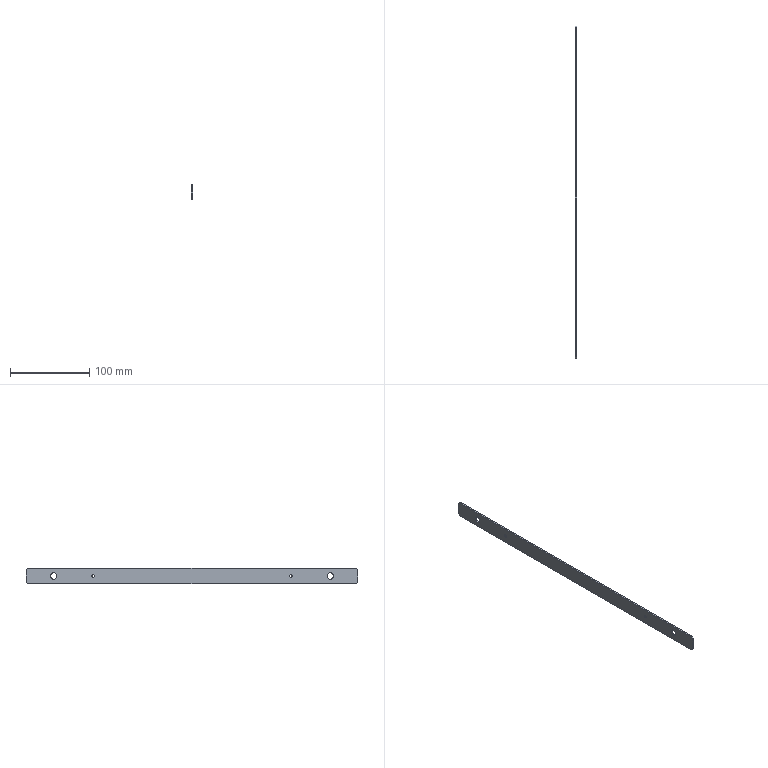Component | SolidWorks | 10-15A-1 | 1 solid | 18 faces | box 2 x 420 x 20 mm | volume 16549 mm3 | plane 10 | cylinder 8 | commonest cylinder face diameters 3.3 x4 8 x4
STEP:
#1=COLOUR_RGB('',0.7922,0.8196,0.9333);
#2=FILL_AREA_STYLE_COLOUR('',#1);
#3=FILL_AREA_STYLE('',(#2));
#4=SURFACE_STYLE_FILL_AREA(#3);
#5=SURFACE_SIDE_STYLE('',(#4));
#6=SURFACE_STYLE_USAGE(.BOTH.,#5);
#7=PRESENTATION_STYLE_ASSIGNMENT((#6));
#8=CARTESIAN_POINT('',(-17.615,14.849,0.8524));
#9=VERTEX_POINT('',#8);
#10=CARTESIAN_POINT('',(-17.615,14.849,0.7224));
#11=VERTEX_POINT('',#10);
#12=CARTESIAN_POINT('',(-17.615,14.849,0.7874));
#13=DIRECTION('',(-1.,0.,0.));
#14=DIRECTION('',(0.,0.,-1.));
#15=AXIS2_PLACEMENT_3D('',#12,#13,#14);
#16=CIRCLE('',#15,0.06496);
#17=EDGE_CURVE('',#9,#11,#16,.T.);
#18=ORIENTED_EDGE('',*,*,#17,.F.);
#19=CARTESIAN_POINT('',(-17.694,14.849,0.8524));
#20=VERTEX_POINT('',#19);
#21=CARTESIAN_POINT('',(-17.694,14.849,0.8524));
#22=DIRECTION('',(-1.,0.,0.));
#23=VECTOR('',#22,39.37);
#24=LINE('',#21,#23);
#25=EDGE_CURVE('',#9,#20,#24,.T.);
#26=ORIENTED_EDGE('',*,*,#25,.T.);
#27=CARTESIAN_POINT('',(-17.694,14.849,0.7224));
#28=VERTEX_POINT('',#27);
#29=CARTESIAN_POINT('',(-17.694,14.849,0.7874));
#30=DIRECTION('',(-1.,0.,0.));
#31=DIRECTION('',(0.,0.,-1.));
#32=AXIS2_PLACEMENT_3D('',#29,#30,#31);
#33=CIRCLE('',#32,0.06496);
#34=EDGE_CURVE('',#20,#28,#33,.T.);
#35=ORIENTED_EDGE('',*,*,#34,.T.);
#36=CARTESIAN_POINT('',(-17.694,14.849,0.7224));
#37=DIRECTION('',(-1.,0.,0.));
#38=VECTOR('',#37,39.37);
#39=LINE('',#36,#38);
#40=EDGE_CURVE('',#11,#28,#39,.T.);
#41=ORIENTED_EDGE('',*,*,#40,.F.);
#42=EDGE_LOOP('',(#18,#26,#35,#41));
#43=FACE_OUTER_BOUND('',#42,.T.);
#44=CARTESIAN_POINT('',(-17.694,14.849,0.7874));
#45=DIRECTION('',(-1.,0.,0.));
#46=DIRECTION('',(0.,0.,-1.));
#47=AXIS2_PLACEMENT_3D('',#44,#45,#46);
#48=CYLINDRICAL_SURFACE('',#47,0.06496);
#49=ADVANCED_FACE('',(#43),#48,.F.);
#50=CARTESIAN_POINT('',(-17.615,24.691,0.8524));
#51=VERTEX_POINT('',#50);
#52=CARTESIAN_POINT('',(-17.615,24.691,0.7224));
#53=VERTEX_POINT('',#52);
#54=CARTESIAN_POINT('',(-17.615,24.691,0.7874));
#55=DIRECTION('',(-1.,0.,0.));
#56=DIRECTION('',(0.,0.,-1.));
#57=AXIS2_PLACEMENT_3D('',#54,#55,#56);
#58=CIRCLE('',#57,0.06496);
#59=EDGE_CURVE('',#51,#53,#58,.T.);
#60=ORIENTED_EDGE('',*,*,#59,.F.);
#61=CARTESIAN_POINT('',(-17.694,24.691,0.8524));
#62=VERTEX_POINT('',#61);
#63=CARTESIAN_POINT('',(-17.694,24.691,0.8524));
#64=DIRECTION('',(-1.,0.,0.));
#65=VECTOR('',#64,39.37);
#66=LINE('',#63,#65);
#67=EDGE_CURVE('',#51,#62,#66,.T.);
#68=ORIENTED_EDGE('',*,*,#67,.T.);
#69=CARTESIAN_POINT('',(-17.694,24.691,0.7224));
#70=VERTEX_POINT('',#69);
#71=CARTESIAN_POINT('',(-17.694,24.691,0.7874));
#72=DIRECTION('',(-1.,0.,0.));
#73=DIRECTION('',(0.,0.,-1.));
#74=AXIS2_PLACEMENT_3D('',#71,#72,#73);
#75=CIRCLE('',#74,0.06496);
#76=EDGE_CURVE('',#62,#70,#75,.T.);
#77=ORIENTED_EDGE('',*,*,#76,.T.);
#78=CARTESIAN_POINT('',(-17.694,24.691,0.7224));
#79=DIRECTION('',(-1.,0.,0.));
#80=VECTOR('',#79,39.37);
#81=LINE('',#78,#80);
#82=EDGE_CURVE('',#53,#70,#81,.T.);
#83=ORIENTED_EDGE('',*,*,#82,.F.);
#84=EDGE_LOOP('',(#60,#68,#77,#83));
#85=FACE_OUTER_BOUND('',#84,.T.);
#86=CARTESIAN_POINT('',(-17.694,24.691,0.7874));
#87=DIRECTION('',(-1.,0.,0.));
#88=DIRECTION('',(0.,0.,-1.));
#89=AXIS2_PLACEMENT_3D('',#86,#87,#88);
#90=CYLINDRICAL_SURFACE('',#89,0.06496);
#91=ADVANCED_FACE('',(#85),#90,.F.);
#92=CARTESIAN_POINT('',(-17.615,26.66,0.9449));
#93=VERTEX_POINT('',#92);
#94=CARTESIAN_POINT('',(-17.615,26.66,0.6299));
#95=VERTEX_POINT('',#94);
#96=CARTESIAN_POINT('',(-17.615,26.66,0.7874));
#97=DIRECTION('',(-1.,0.,0.));
#98=DIRECTION('',(0.,0.,-1.));
#99=AXIS2_PLACEMENT_3D('',#96,#97,#98);
#100=CIRCLE('',#99,0.1575);
#101=EDGE_CURVE('',#93,#95,#100,.T.);
#102=ORIENTED_EDGE('',*,*,#101,.F.);
#103=CARTESIAN_POINT('',(-17.694,26.66,0.9449));
#104=VERTEX_POINT('',#103);
#105=CARTESIAN_POINT('',(-17.3,26.66,0.9449));
#106=DIRECTION('',(-1.,0.,0.));
#107=VECTOR('',#106,39.37);
#108=LINE('',#105,#107);
#109=EDGE_CURVE('',#93,#104,#108,.T.);
#110=ORIENTED_EDGE('',*,*,#109,.T.);
#111=CARTESIAN_POINT('',(-17.694,26.66,0.6299));
#112=VERTEX_POINT('',#111);
#113=CARTESIAN_POINT('',(-17.694,26.66,0.7874));
#114=DIRECTION('',(-1.,0.,0.));
#115=DIRECTION('',(0.,0.,-1.));
#116=AXIS2_PLACEMENT_3D('',#113,#114,#115);
#117=CIRCLE('',#116,0.1575);
#118=EDGE_CURVE('',#104,#112,#117,.T.);
#119=ORIENTED_EDGE('',*,*,#118,.T.);
#120=CARTESIAN_POINT('',(-17.3,26.66,0.6299));
#121=DIRECTION('',(-1.,0.,0.));
#122=VECTOR('',#121,39.37);
#123=LINE('',#120,#122);
#124=EDGE_CURVE('',#95,#112,#123,.T.);
#125=ORIENTED_EDGE('',*,*,#124,.F.);
#126=EDGE_LOOP('',(#102,#110,#119,#125));
#127=FACE_OUTER_BOUND('',#126,.T.);
#128=CARTESIAN_POINT('',(-17.3,26.66,0.7874));
#129=DIRECTION('',(-1.,0.,0.));
#130=DIRECTION('',(0.,0.,-1.));
#131=AXIS2_PLACEMENT_3D('',#128,#129,#130);
#132=CYLINDRICAL_SURFACE('',#131,0.1575);
#133=ADVANCED_FACE('',(#127),#132,.F.);
#134=CARTESIAN_POINT('',(-17.615,12.88,0.9449));
#135=VERTEX_POINT('',#134);
#136=CARTESIAN_POINT('',(-17.615,12.88,0.6299));
#137=VERTEX_POINT('',#136);
#138=CARTESIAN_POINT('',(-17.615,12.88,0.7874));
#139=DIRECTION('',(-1.,0.,0.));
#140=DIRECTION('',(0.,0.,-1.));
#141=AXIS2_PLACEMENT_3D('',#138,#139,#140);
#142=CIRCLE('',#141,0.1575);
#143=EDGE_CURVE('',#135,#137,#142,.T.);
#144=ORIENTED_EDGE('',*,*,#143,.F.);
#145=CARTESIAN_POINT('',(-17.694,12.88,0.9449));
#146=VERTEX_POINT('',#145);
#147=CARTESIAN_POINT('',(-17.3,12.88,0.9449));
#148=DIRECTION('',(-1.,0.,0.));
#149=VECTOR('',#148,39.37);
#150=LINE('',#147,#149);
#151=EDGE_CURVE('',#135,#146,#150,.T.);
#152=ORIENTED_EDGE('',*,*,#151,.T.);
#153=CARTESIAN_POINT('',(-17.694,12.88,0.6299));
#154=VERTEX_POINT('',#153);
#155=CARTESIAN_POINT('',(-17.694,12.88,0.7874));
#156=DIRECTION('',(-1.,0.,0.));
#157=DIRECTION('',(0.,0.,-1.));
#158=AXIS2_PLACEMENT_3D('',#155,#156,#157);
#159=CIRCLE('',#158,0.1575);
#160=EDGE_CURVE('',#146,#154,#159,.T.);
#161=ORIENTED_EDGE('',*,*,#160,.T.);
#162=CARTESIAN_POINT('',(-17.3,12.88,0.6299));
#163=DIRECTION('',(-1.,0.,0.));
#164=VECTOR('',#163,39.37);
#165=LINE('',#162,#164);
#166=EDGE_CURVE('',#137,#154,#165,.T.);
#167=ORIENTED_EDGE('',*,*,#166,.F.);
#168=EDGE_LOOP('',(#144,#152,#161,#167));
#169=FACE_OUTER_BOUND('',#168,.T.);
#170=CARTESIAN_POINT('',(-17.3,12.88,0.7874));
#171=DIRECTION('',(-1.,0.,0.));
#172=DIRECTION('',(0.,0.,-1.));
#173=AXIS2_PLACEMENT_3D('',#170,#171,#172);
#174=CYLINDRICAL_SURFACE('',#173,0.1575);
#175=ADVANCED_FACE('',(#169),#174,.F.);
#176=CARTESIAN_POINT('',(-17.615,11.581,1.181));
#177=VERTEX_POINT('',#176);
#178=CARTESIAN_POINT('',(-17.615,27.959,1.181));
#179=VERTEX_POINT('',#178);
#180=CARTESIAN_POINT('',(-17.615,11.502,1.181));
#181=DIRECTION('',(0.,1.,-0.));
#182=VECTOR('',#181,39.37);
#183=LINE('',#180,#182);
#184=EDGE_CURVE('',#177,#179,#183,.T.);
#185=ORIENTED_EDGE('',*,*,#184,.T.);
#186=CARTESIAN_POINT('',(-17.694,27.959,1.181));
#187=VERTEX_POINT('',#186);
#188=CARTESIAN_POINT('',(-17.694,27.959,1.181));
#189=DIRECTION('',(-1.,0.,0.));
#190=VECTOR('',#189,39.37);
#191=LINE('',#188,#190);
#192=EDGE_CURVE('',#179,#187,#191,.T.);
#193=ORIENTED_EDGE('',*,*,#192,.T.);
#194=CARTESIAN_POINT('',(-17.694,11.581,1.181));
#195=VERTEX_POINT('',#194);
#196=CARTESIAN_POINT('',(-17.694,11.502,1.181));
#197=DIRECTION('',(0.,1.,-0.));
#198=VECTOR('',#197,39.37);
#199=LINE('',#196,#198);
#200=EDGE_CURVE('',#195,#187,#199,.T.);
#201=ORIENTED_EDGE('',*,*,#200,.F.);
#202=CARTESIAN_POINT('',(-17.694,11.581,1.181));
#203=DIRECTION('',(1.,-0.,-0.));
#204=VECTOR('',#203,39.37);
#205=LINE('',#202,#204);
#206=EDGE_CURVE('',#195,#177,#205,.T.);
#207=ORIENTED_EDGE('',*,*,#206,.T.);
#208=EDGE_LOOP('',(#185,#193,#201,#207));
#209=FACE_OUTER_BOUND('',#208,.T.);
#210=CARTESIAN_POINT('',(-17.694,11.502,1.181));
#211=DIRECTION('',(-0.,-0.,-1.));
#212=DIRECTION('',(-0.,-1.,0.));
#213=AXIS2_PLACEMENT_3D('',#210,#211,#212);
#214=PLANE('',#213);
#215=ADVANCED_FACE('',(#209),#214,.F.);
#216=CARTESIAN_POINT('',(-17.694,28.038,1.102));
#217=VERTEX_POINT('',#216);
#218=CARTESIAN_POINT('',(-17.694,28.038,0.4724));
#219=VERTEX_POINT('',#218);
#220=CARTESIAN_POINT('',(-17.694,28.038,1.181));
#221=DIRECTION('',(-0.,0.,-1.));
#222=VECTOR('',#221,39.37);
#223=LINE('',#220,#222);
#224=EDGE_CURVE('',#217,#219,#223,.T.);
#225=ORIENTED_EDGE('',*,*,#224,.F.);
#226=CARTESIAN_POINT('',(-17.615,28.038,1.102));
#227=VERTEX_POINT('',#226);
#228=CARTESIAN_POINT('',(-17.694,28.038,1.102));
#229=DIRECTION('',(1.,-0.,-0.));
#230=VECTOR('',#229,39.37);
#231=LINE('',#228,#230);
#232=EDGE_CURVE('',#217,#227,#231,.T.);
#233=ORIENTED_EDGE('',*,*,#232,.T.);
#234=CARTESIAN_POINT('',(-17.615,28.038,0.4724));
#235=VERTEX_POINT('',#234);
#236=CARTESIAN_POINT('',(-17.615,28.038,1.181));
#237=DIRECTION('',(-0.,0.,-1.));
#238=VECTOR('',#237,39.37);
#239=LINE('',#236,#238);
#240=EDGE_CURVE('',#227,#235,#239,.T.);
#241=ORIENTED_EDGE('',*,*,#240,.T.);
#242=CARTESIAN_POINT('',(-17.694,28.038,0.4724));
#243=DIRECTION('',(-1.,0.,0.));
#244=VECTOR('',#243,39.37);
#245=LINE('',#242,#244);
#246=EDGE_CURVE('',#235,#219,#245,.T.);
#247=ORIENTED_EDGE('',*,*,#246,.T.);
#248=EDGE_LOOP('',(#225,#233,#241,#247));
#249=FACE_OUTER_BOUND('',#248,.T.);
#250=CARTESIAN_POINT('',(-17.694,28.038,1.181));
#251=DIRECTION('',(-0.,-1.,-0.));
#252=DIRECTION('',(-1.,0.,0.));
#253=AXIS2_PLACEMENT_3D('',#250,#251,#252);
#254=PLANE('',#253);
#255=ADVANCED_FACE('',(#249),#254,.F.);
#256=CARTESIAN_POINT('',(-17.694,27.959,0.3937));
#257=VERTEX_POINT('',#256);
#258=CARTESIAN_POINT('',(-17.694,11.581,0.3937));
#259=VERTEX_POINT('',#258);
#260=CARTESIAN_POINT('',(-17.694,11.502,0.3937));
#261=DIRECTION('',(-0.,-1.,0.));
#262=VECTOR('',#261,39.37);
#263=LINE('',#260,#262);
#264=EDGE_CURVE('',#257,#259,#263,.T.);
#265=ORIENTED_EDGE('',*,*,#264,.F.);
#266=CARTESIAN_POINT('',(-17.615,27.959,0.3937));
#267=VERTEX_POINT('',#266);
#268=CARTESIAN_POINT('',(-17.694,27.959,0.3937));
#269=DIRECTION('',(1.,-0.,-0.));
#270=VECTOR('',#269,39.37);
#271=LINE('',#268,#270);
#272=EDGE_CURVE('',#257,#267,#271,.T.);
#273=ORIENTED_EDGE('',*,*,#272,.T.);
#274=CARTESIAN_POINT('',(-17.615,11.581,0.3937));
#275=VERTEX_POINT('',#274);
#276=CARTESIAN_POINT('',(-17.615,11.502,0.3937));
#277=DIRECTION('',(-0.,-1.,0.));
#278=VECTOR('',#277,39.37);
#279=LINE('',#276,#278);
#280=EDGE_CURVE('',#267,#275,#279,.T.);
#281=ORIENTED_EDGE('',*,*,#280,.T.);
#282=CARTESIAN_POINT('',(-17.694,11.581,0.3937));
#283=DIRECTION('',(-1.,0.,0.));
#284=VECTOR('',#283,39.37);
#285=LINE('',#282,#284);
#286=EDGE_CURVE('',#275,#259,#285,.T.);
#287=ORIENTED_EDGE('',*,*,#286,.T.);
#288=EDGE_LOOP('',(#265,#273,#281,#287));
#289=FACE_OUTER_BOUND('',#288,.T.);
#290=CARTESIAN_POINT('',(-17.694,11.502,0.3937));
#291=DIRECTION('',(0.,0.,1.));
#292=DIRECTION('',(0.,1.,-0.));
#293=AXIS2_PLACEMENT_3D('',#290,#291,#292);
#294=PLANE('',#293);
#295=ADVANCED_FACE('',(#289),#294,.F.);
#296=CARTESIAN_POINT('',(-17.615,11.502,0.4724));
#297=VERTEX_POINT('',#296);
#298=CARTESIAN_POINT('',(-17.615,11.502,1.102));
#299=VERTEX_POINT('',#298);
#300=CARTESIAN_POINT('',(-17.615,11.502,1.181));
#301=DIRECTION('',(0.,0.,1.));
#302=VECTOR('',#301,39.37);
#303=LINE('',#300,#302);
#304=EDGE_CURVE('',#297,#299,#303,.T.);
#305=ORIENTED_EDGE('',*,*,#304,.T.);
#306=CARTESIAN_POINT('',(-17.694,11.502,1.102));
#307=VERTEX_POINT('',#306);
#308=CARTESIAN_POINT('',(-17.694,11.502,1.102));
#309=DIRECTION('',(-1.,0.,0.));
#310=VECTOR('',#309,39.37);
#311=LINE('',#308,#310);
#312=EDGE_CURVE('',#299,#307,#311,.T.);
#313=ORIENTED_EDGE('',*,*,#312,.T.);
#314=CARTESIAN_POINT('',(-17.694,11.502,0.4724));
#315=VERTEX_POINT('',#314);
#316=CARTESIAN_POINT('',(-17.694,11.502,1.181));
#317=DIRECTION('',(0.,0.,1.));
#318=VECTOR('',#317,39.37);
#319=LINE('',#316,#318);
#320=EDGE_CURVE('',#315,#307,#319,.T.);
#321=ORIENTED_EDGE('',*,*,#320,.F.);
#322=CARTESIAN_POINT('',(-17.694,11.502,0.4724));
#323=DIRECTION('',(1.,-0.,-0.));
#324=VECTOR('',#323,39.37);
#325=LINE('',#322,#324);
#326=EDGE_CURVE('',#315,#297,#325,.T.);
#327=ORIENTED_EDGE('',*,*,#326,.T.);
#328=EDGE_LOOP('',(#305,#313,#321,#327));
#329=FACE_OUTER_BOUND('',#328,.T.);
#330=CARTESIAN_POINT('',(-17.694,11.502,1.181));
#331=DIRECTION('',(0.,1.,0.));
#332=DIRECTION('',(1.,-0.,-0.));
#333=AXIS2_PLACEMENT_3D('',#330,#331,#332);
#334=PLANE('',#333);
#335=ADVANCED_FACE('',(#329),#334,.F.);
#336=CARTESIAN_POINT('',(-17.694,14.849,0.7874));
#337=DIRECTION('',(-1.,0.,0.));
#338=DIRECTION('',(0.,0.,-1.));
#339=AXIS2_PLACEMENT_3D('',#336,#337,#338);
#340=CIRCLE('',#339,0.06496);
#341=EDGE_CURVE('',#28,#20,#340,.T.);
#342=ORIENTED_EDGE('',*,*,#341,.F.);
#343=ORIENTED_EDGE('',*,*,#34,.F.);
#344=EDGE_LOOP('',(#342,#343));
#345=FACE_BOUND('',#344,.T.);
#346=CARTESIAN_POINT('',(-17.694,24.691,0.7874));
#347=DIRECTION('',(-1.,0.,0.));
#348=DIRECTION('',(0.,0.,-1.));
#349=AXIS2_PLACEMENT_3D('',#346,#347,#348);
#350=CIRCLE('',#349,0.06496);
#351=EDGE_CURVE('',#70,#62,#350,.T.);
#352=ORIENTED_EDGE('',*,*,#351,.F.);
#353=ORIENTED_EDGE('',*,*,#76,.F.);
#354=EDGE_LOOP('',(#352,#353));
#355=FACE_BOUND('',#354,.T.);
#356=CARTESIAN_POINT('',(-17.694,26.66,0.7874));
#357=DIRECTION('',(-1.,0.,0.));
#358=DIRECTION('',(0.,0.,-1.));
#359=AXIS2_PLACEMENT_3D('',#356,#357,#358);
#360=CIRCLE('',#359,0.1575);
#361=EDGE_CURVE('',#112,#104,#360,.T.);
#362=ORIENTED_EDGE('',*,*,#361,.F.);
#363=ORIENTED_EDGE('',*,*,#118,.F.);
#364=EDGE_LOOP('',(#362,#363));
#365=FACE_BOUND('',#364,.T.);
#366=CARTESIAN_POINT('',(-17.694,12.88,0.7874));
#367=DIRECTION('',(-1.,0.,0.));
#368=DIRECTION('',(0.,0.,-1.));
#369=AXIS2_PLACEMENT_3D('',#366,#367,#368);
#370=CIRCLE('',#369,0.1575);
#371=EDGE_CURVE('',#154,#146,#370,.T.);
#372=ORIENTED_EDGE('',*,*,#371,.F.);
#373=ORIENTED_EDGE('',*,*,#160,.F.);
#374=EDGE_LOOP('',(#372,#373));
#375=FACE_BOUND('',#374,.T.);
#376=ORIENTED_EDGE('',*,*,#200,.T.);
#377=CARTESIAN_POINT('',(-17.694,27.998,1.142));
#378=DIRECTION('',(0.,0.7071,-0.7071));
#379=VECTOR('',#378,39.37);
#380=LINE('',#377,#379);
#381=EDGE_CURVE('',#187,#217,#380,.T.);
#382=ORIENTED_EDGE('',*,*,#381,.T.);
#383=ORIENTED_EDGE('',*,*,#224,.T.);
#384=CARTESIAN_POINT('',(-17.694,28.392,0.8268));
#385=DIRECTION('',(-0.,-0.7071,-0.7071));
#386=VECTOR('',#385,39.37);
#387=LINE('',#384,#386);
#388=EDGE_CURVE('',#219,#257,#387,.T.);
#389=ORIENTED_EDGE('',*,*,#388,.T.);
#390=ORIENTED_EDGE('',*,*,#264,.T.);
#391=CARTESIAN_POINT('',(-17.694,19.416,-7.441));
#392=DIRECTION('',(-0.,-0.7071,0.7071));
#393=VECTOR('',#392,39.37);
#394=LINE('',#391,#393);
#395=EDGE_CURVE('',#259,#315,#394,.T.);
#396=ORIENTED_EDGE('',*,*,#395,.T.);
#397=ORIENTED_EDGE('',*,*,#320,.T.);
#398=CARTESIAN_POINT('',(-17.694,19.809,9.409));
#399=DIRECTION('',(0.,0.7071,0.7071));
#400=VECTOR('',#399,39.37);
#401=LINE('',#398,#400);
#402=EDGE_CURVE('',#307,#195,#401,.T.);
#403=ORIENTED_EDGE('',*,*,#402,.T.);
#404=EDGE_LOOP('',(#376,#382,#383,#389,#390,#396,#397,#403));
#405=FACE_OUTER_BOUND('',#404,.T.);
#406=CARTESIAN_POINT('',(-17.694,28.038,1.181));
#407=DIRECTION('',(-1.,0.,0.));
#408=DIRECTION('',(-0.,0.,-1.));
#409=AXIS2_PLACEMENT_3D('',#406,#407,#408);
#410=PLANE('',#409);
#411=ADVANCED_FACE('',(#345,#355,#365,#375,#405),#410,.T.);
#412=CARTESIAN_POINT('',(-17.615,14.849,0.7874));
#413=DIRECTION('',(-1.,0.,0.));
#414=DIRECTION('',(0.,0.,-1.));
#415=AXIS2_PLACEMENT_3D('',#412,#413,#414);
#416=CIRCLE('',#415,0.06496);
#417=EDGE_CURVE('',#11,#9,#416,.T.);
#418=ORIENTED_EDGE('',*,*,#417,.T.);
#419=ORIENTED_EDGE('',*,*,#17,.T.);
#420=EDGE_LOOP('',(#418,#419));
#421=FACE_BOUND('',#420,.T.);
#422=CARTESIAN_POINT('',(-17.615,24.691,0.7874));
#423=DIRECTION('',(-1.,0.,0.));
#424=DIRECTION('',(0.,0.,-1.));
#425=AXIS2_PLACEMENT_3D('',#422,#423,#424);
#426=CIRCLE('',#425,0.06496);
#427=EDGE_CURVE('',#53,#51,#426,.T.);
#428=ORIENTED_EDGE('',*,*,#427,.T.);
#429=ORIENTED_EDGE('',*,*,#59,.T.);
#430=EDGE_LOOP('',(#428,#429));
#431=FACE_BOUND('',#430,.T.);
#432=CARTESIAN_POINT('',(-17.615,26.66,0.7874));
#433=DIRECTION('',(-1.,0.,0.));
#434=DIRECTION('',(0.,0.,-1.));
#435=AXIS2_PLACEMENT_3D('',#432,#433,#434);
#436=CIRCLE('',#435,0.1575);
#437=EDGE_CURVE('',#95,#93,#436,.T.);
#438=ORIENTED_EDGE('',*,*,#437,.T.);
#439=ORIENTED_EDGE('',*,*,#101,.T.);
#440=EDGE_LOOP('',(#438,#439));
#441=FACE_BOUND('',#440,.T.);
#442=CARTESIAN_POINT('',(-17.615,12.88,0.7874));
#443=DIRECTION('',(-1.,0.,0.));
#444=DIRECTION('',(0.,0.,-1.));
#445=AXIS2_PLACEMENT_3D('',#442,#443,#444);
#446=CIRCLE('',#445,0.1575);
#447=EDGE_CURVE('',#137,#135,#446,.T.);
#448=ORIENTED_EDGE('',*,*,#447,.T.);
#449=ORIENTED_EDGE('',*,*,#143,.T.);
#450=EDGE_LOOP('',(#448,#449));
#451=FACE_BOUND('',#450,.T.);
#452=ORIENTED_EDGE('',*,*,#240,.F.);
#453=CARTESIAN_POINT('',(-17.615,28.038,1.102));
#454=DIRECTION('',(-0.,-0.7071,0.7071));
#455=VECTOR('',#454,39.37);
#456=LINE('',#453,#455);
#457=EDGE_CURVE('',#227,#179,#456,.T.);
#458=ORIENTED_EDGE('',*,*,#457,.T.);
#459=ORIENTED_EDGE('',*,*,#184,.F.);
#460=CARTESIAN_POINT('',(-17.615,11.581,1.181));
#461=DIRECTION('',(-0.,-0.7071,-0.7071));
#462=VECTOR('',#461,39.37);
#463=LINE('',#460,#462);
#464=EDGE_CURVE('',#177,#299,#463,.T.);
#465=ORIENTED_EDGE('',*,*,#464,.T.);
#466=ORIENTED_EDGE('',*,*,#304,.F.);
#467=CARTESIAN_POINT('',(-17.615,11.502,0.4724));
#468=DIRECTION('',(0.,0.7071,-0.7071));
#469=VECTOR('',#468,39.37);
#470=LINE('',#467,#469);
#471=EDGE_CURVE('',#297,#275,#470,.T.);
#472=ORIENTED_EDGE('',*,*,#471,.T.);
#473=ORIENTED_EDGE('',*,*,#280,.F.);
#474=CARTESIAN_POINT('',(-17.615,27.959,0.3937));
#475=DIRECTION('',(0.,0.7071,0.7071));
#476=VECTOR('',#475,39.37);
#477=LINE('',#474,#476);
#478=EDGE_CURVE('',#267,#235,#477,.T.);
#479=ORIENTED_EDGE('',*,*,#478,.T.);
#480=EDGE_LOOP('',(#452,#458,#459,#465,#466,#472,#473,#479));
#481=FACE_OUTER_BOUND('',#480,.T.);
#482=CARTESIAN_POINT('',(-17.615,28.038,1.181));
#483=DIRECTION('',(-1.,0.,0.));
#484=DIRECTION('',(-0.,0.,-1.));
#485=AXIS2_PLACEMENT_3D('',#482,#483,#484);
#486=PLANE('',#485);
#487=ADVANCED_FACE('',(#421,#431,#441,#451,#481),#486,.F.);
#488=ORIENTED_EDGE('',*,*,#151,.F.);
#489=ORIENTED_EDGE('',*,*,#447,.F.);
#490=ORIENTED_EDGE('',*,*,#166,.T.);
#491=ORIENTED_EDGE('',*,*,#371,.T.);
#492=EDGE_LOOP('',(#488,#489,#490,#491));
#493=FACE_OUTER_BOUND('',#492,.T.);
#494=CARTESIAN_POINT('',(-17.3,12.88,0.7874));
#495=DIRECTION('',(-1.,0.,0.));
#496=DIRECTION('',(0.,0.,-1.));
#497=AXIS2_PLACEMENT_3D('',#494,#495,#496);
#498=CYLINDRICAL_SURFACE('',#497,0.1575);
#499=ADVANCED_FACE('',(#493),#498,.F.);
#500=ORIENTED_EDGE('',*,*,#109,.F.);
#501=ORIENTED_EDGE('',*,*,#437,.F.);
#502=ORIENTED_EDGE('',*,*,#124,.T.);
#503=ORIENTED_EDGE('',*,*,#361,.T.);
#504=EDGE_LOOP('',(#500,#501,#502,#503));
#505=FACE_OUTER_BOUND('',#504,.T.);
#506=CARTESIAN_POINT('',(-17.3,26.66,0.7874));
#507=DIRECTION('',(-1.,0.,0.));
#508=DIRECTION('',(0.,0.,-1.));
#509=AXIS2_PLACEMENT_3D('',#506,#507,#508);
#510=CYLINDRICAL_SURFACE('',#509,0.1575);
#511=ADVANCED_FACE('',(#505),#510,.F.);
#512=ORIENTED_EDGE('',*,*,#381,.F.);
#513=ORIENTED_EDGE('',*,*,#192,.F.);
#514=ORIENTED_EDGE('',*,*,#457,.F.);
#515=ORIENTED_EDGE('',*,*,#232,.F.);
#516=EDGE_LOOP('',(#512,#513,#514,#515));
#517=FACE_OUTER_BOUND('',#516,.T.);
#518=CARTESIAN_POINT('',(-17.694,28.038,1.102));
#519=DIRECTION('',(-0.,-0.7071,-0.7071));
#520=DIRECTION('',(-0.,-0.7071,0.7071));
#521=AXIS2_PLACEMENT_3D('',#518,#519,#520);
#522=PLANE('',#521);
#523=ADVANCED_FACE('',(#517),#522,.F.);
#524=ORIENTED_EDGE('',*,*,#388,.F.);
#525=ORIENTED_EDGE('',*,*,#246,.F.);
#526=ORIENTED_EDGE('',*,*,#478,.F.);
#527=ORIENTED_EDGE('',*,*,#272,.F.);
#528=EDGE_LOOP('',(#524,#525,#526,#527));
#529=FACE_OUTER_BOUND('',#528,.T.);
#530=CARTESIAN_POINT('',(-17.694,27.959,0.3937));
#531=DIRECTION('',(-0.,-0.7071,0.7071));
#532=DIRECTION('',(0.,0.7071,0.7071));
#533=AXIS2_PLACEMENT_3D('',#530,#531,#532);
#534=PLANE('',#533);
#535=ADVANCED_FACE('',(#529),#534,.F.);
#536=ORIENTED_EDGE('',*,*,#402,.F.);
#537=ORIENTED_EDGE('',*,*,#312,.F.);
#538=ORIENTED_EDGE('',*,*,#464,.F.);
#539=ORIENTED_EDGE('',*,*,#206,.F.);
#540=EDGE_LOOP('',(#536,#537,#538,#539));
#541=FACE_OUTER_BOUND('',#540,.T.);
#542=CARTESIAN_POINT('',(-17.694,11.581,1.181));
#543=DIRECTION('',(0.,0.7071,-0.7071));
#544=DIRECTION('',(-0.,-0.7071,-0.7071));
#545=AXIS2_PLACEMENT_3D('',#542,#543,#544);
#546=PLANE('',#545);
#547=ADVANCED_FACE('',(#541),#546,.F.);
#548=ORIENTED_EDGE('',*,*,#395,.F.);
#549=ORIENTED_EDGE('',*,*,#286,.F.);
#550=ORIENTED_EDGE('',*,*,#471,.F.);
#551=ORIENTED_EDGE('',*,*,#326,.F.);
#552=EDGE_LOOP('',(#548,#549,#550,#551));
#553=FACE_OUTER_BOUND('',#552,.T.);
#554=CARTESIAN_POINT('',(-17.694,11.502,0.4724));
#555=DIRECTION('',(0.,0.7071,0.7071));
#556=DIRECTION('',(0.,0.7071,-0.7071));
#557=AXIS2_PLACEMENT_3D('',#554,#555,#556);
#558=PLANE('',#557);
#559=ADVANCED_FACE('',(#553),#558,.F.);
#560=ORIENTED_EDGE('',*,*,#67,.F.);
#561=ORIENTED_EDGE('',*,*,#427,.F.);
#562=ORIENTED_EDGE('',*,*,#82,.T.);
#563=ORIENTED_EDGE('',*,*,#351,.T.);
#564=EDGE_LOOP('',(#560,#561,#562,#563));
#565=FACE_OUTER_BOUND('',#564,.T.);
#566=CARTESIAN_POINT('',(-17.694,24.691,0.7874));
#567=DIRECTION('',(-1.,0.,0.));
#568=DIRECTION('',(0.,0.,-1.));
#569=AXIS2_PLACEMENT_3D('',#566,#567,#568);
#570=CYLINDRICAL_SURFACE('',#569,0.06496);
#571=ADVANCED_FACE('',(#565),#570,.F.);
#572=ORIENTED_EDGE('',*,*,#25,.F.);
#573=ORIENTED_EDGE('',*,*,#417,.F.);
#574=ORIENTED_EDGE('',*,*,#40,.T.);
#575=ORIENTED_EDGE('',*,*,#341,.T.);
#576=EDGE_LOOP('',(#572,#573,#574,#575));
#577=FACE_OUTER_BOUND('',#576,.T.);
#578=CARTESIAN_POINT('',(-17.694,14.849,0.7874));
#579=DIRECTION('',(-1.,0.,0.));
#580=DIRECTION('',(0.,0.,-1.));
#581=AXIS2_PLACEMENT_3D('',#578,#579,#580);
#582=CYLINDRICAL_SURFACE('',#581,0.06496);
#583=ADVANCED_FACE('',(#577),#582,.F.);
#584=CLOSED_SHELL('',(#49,#91,#133,#175,#215,#255,#295,#335,#411,#487,#499,#511,#523,#535,#547,#559,#571,#583));
#585=MANIFOLD_SOLID_BREP('',#584);
#586=STYLED_ITEM('',(#7),#585);
#587=PRESENTATION_LAYER_ASSIGNMENT('','',(#586));
#588=(LENGTH_UNIT()NAMED_UNIT(*)SI_UNIT($,.METRE.));
#589=LENGTH_MEASURE_WITH_UNIT(LENGTH_MEASURE(0.0254),#588);
#590=DIMENSIONAL_EXPONENTS(1.,0.,0.,0.,0.,0.,0.);
#591=(CONVERSION_BASED_UNIT('',#589)LENGTH_UNIT()NAMED_UNIT(#590));
#592=UNCERTAINTY_MEASURE_WITH_UNIT(LENGTH_MEASURE(0.00001),#591,'','');
#593=(NAMED_UNIT(*)PLANE_ANGLE_UNIT()SI_UNIT($,.RADIAN.));
#594=(NAMED_UNIT(*)SI_UNIT($,.STERADIAN.)SOLID_ANGLE_UNIT());
#595=(GEOMETRIC_REPRESENTATION_CONTEXT(3)GLOBAL_UNCERTAINTY_ASSIGNED_CONTEXT((#592))GLOBAL_UNIT_ASSIGNED_CONTEXT((#591,#593,#594))REPRESENTATION_CONTEXT('',''));
#596=MECHANICAL_DESIGN_GEOMETRIC_PRESENTATION_REPRESENTATION('',(#586),#595);
#597=CARTESIAN_POINT('',(0.,0.,0.));
#598=DIRECTION('',(0.,0.,1.));
#599=DIRECTION('',(1.,0.,0.));
#600=AXIS2_PLACEMENT_3D('',#597,#598,#599);
#601=(LENGTH_UNIT()NAMED_UNIT(*)SI_UNIT($,.METRE.));
#602=LENGTH_MEASURE_WITH_UNIT(LENGTH_MEASURE(0.0254),#601);
#603=DIMENSIONAL_EXPONENTS(1.,0.,0.,0.,0.,0.,0.);
#604=(CONVERSION_BASED_UNIT('',#602)LENGTH_UNIT()NAMED_UNIT(#603));
#605=UNCERTAINTY_MEASURE_WITH_UNIT(LENGTH_MEASURE(0.00001),#604,'','');
#606=(NAMED_UNIT(*)PLANE_ANGLE_UNIT()SI_UNIT($,.RADIAN.));
#607=(NAMED_UNIT(*)SI_UNIT($,.STERADIAN.)SOLID_ANGLE_UNIT());
#608=(GEOMETRIC_REPRESENTATION_CONTEXT(3)GLOBAL_UNCERTAINTY_ASSIGNED_CONTEXT((#605))GLOBAL_UNIT_ASSIGNED_CONTEXT((#604,#606,#607))REPRESENTATION_CONTEXT('',''));
#609=ADVANCED_BREP_SHAPE_REPRESENTATION('',(#585,#600),#608);